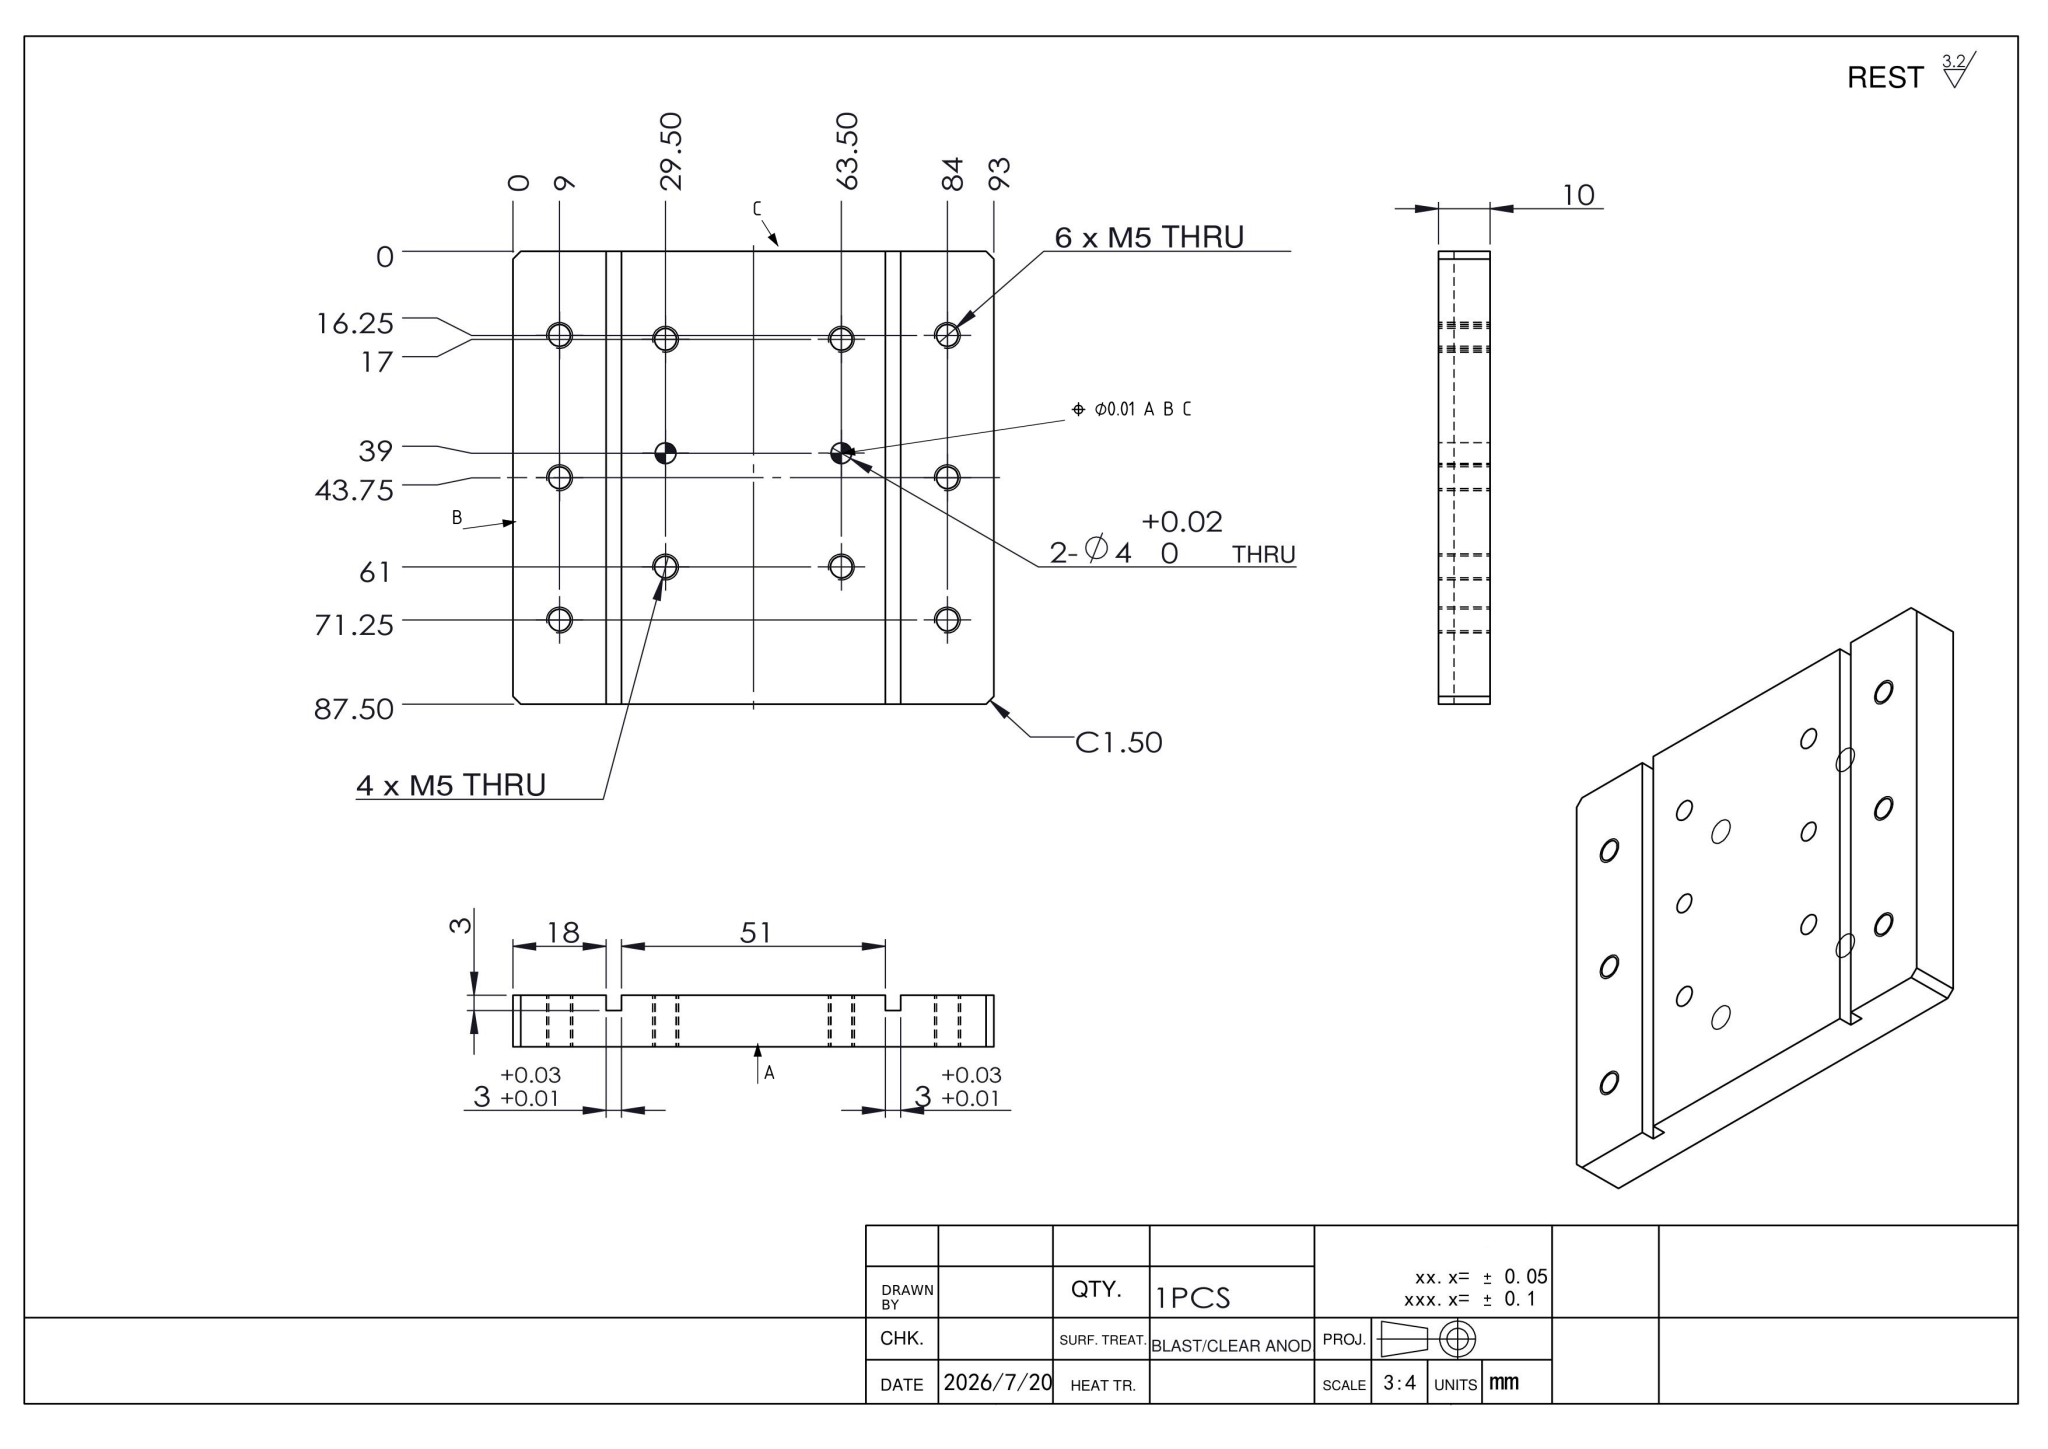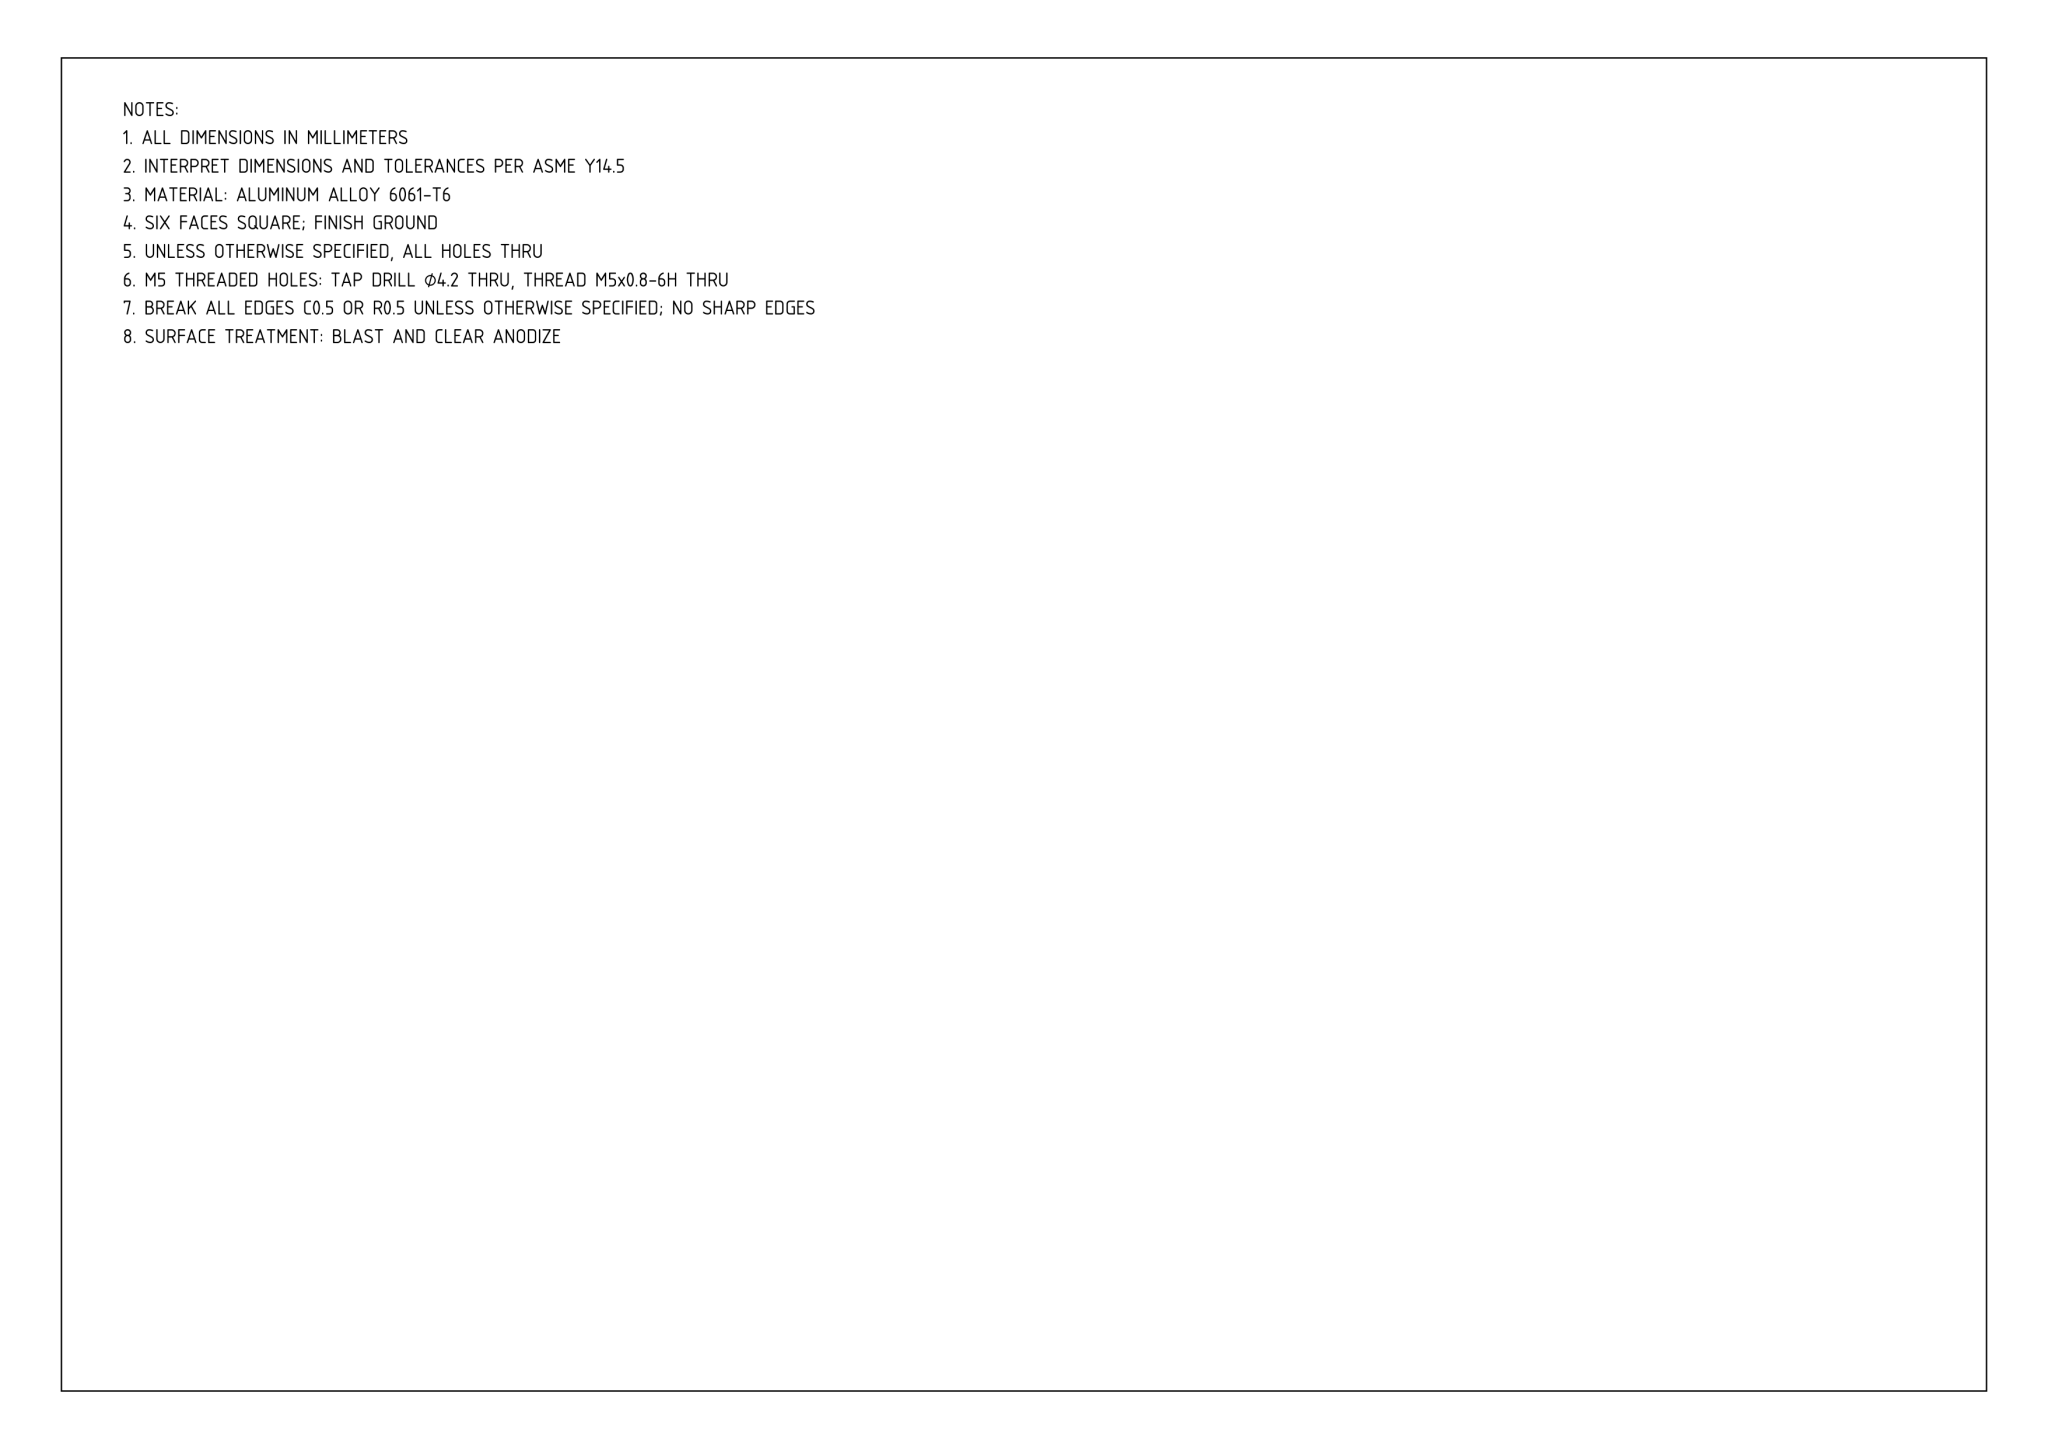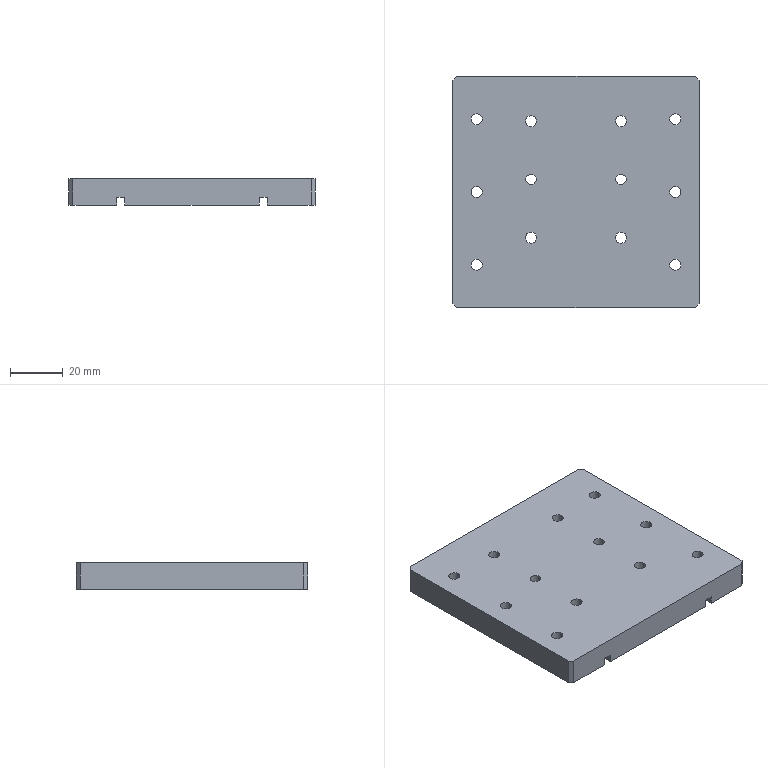Part | NX | mm | 1 solid | 42 faces | box 93 x 87.5 x 10 mm | volume 78118 mm3 | cylinder 24 | plane 18 | commonest cylinder face diameters 4.2 x20 4 x4